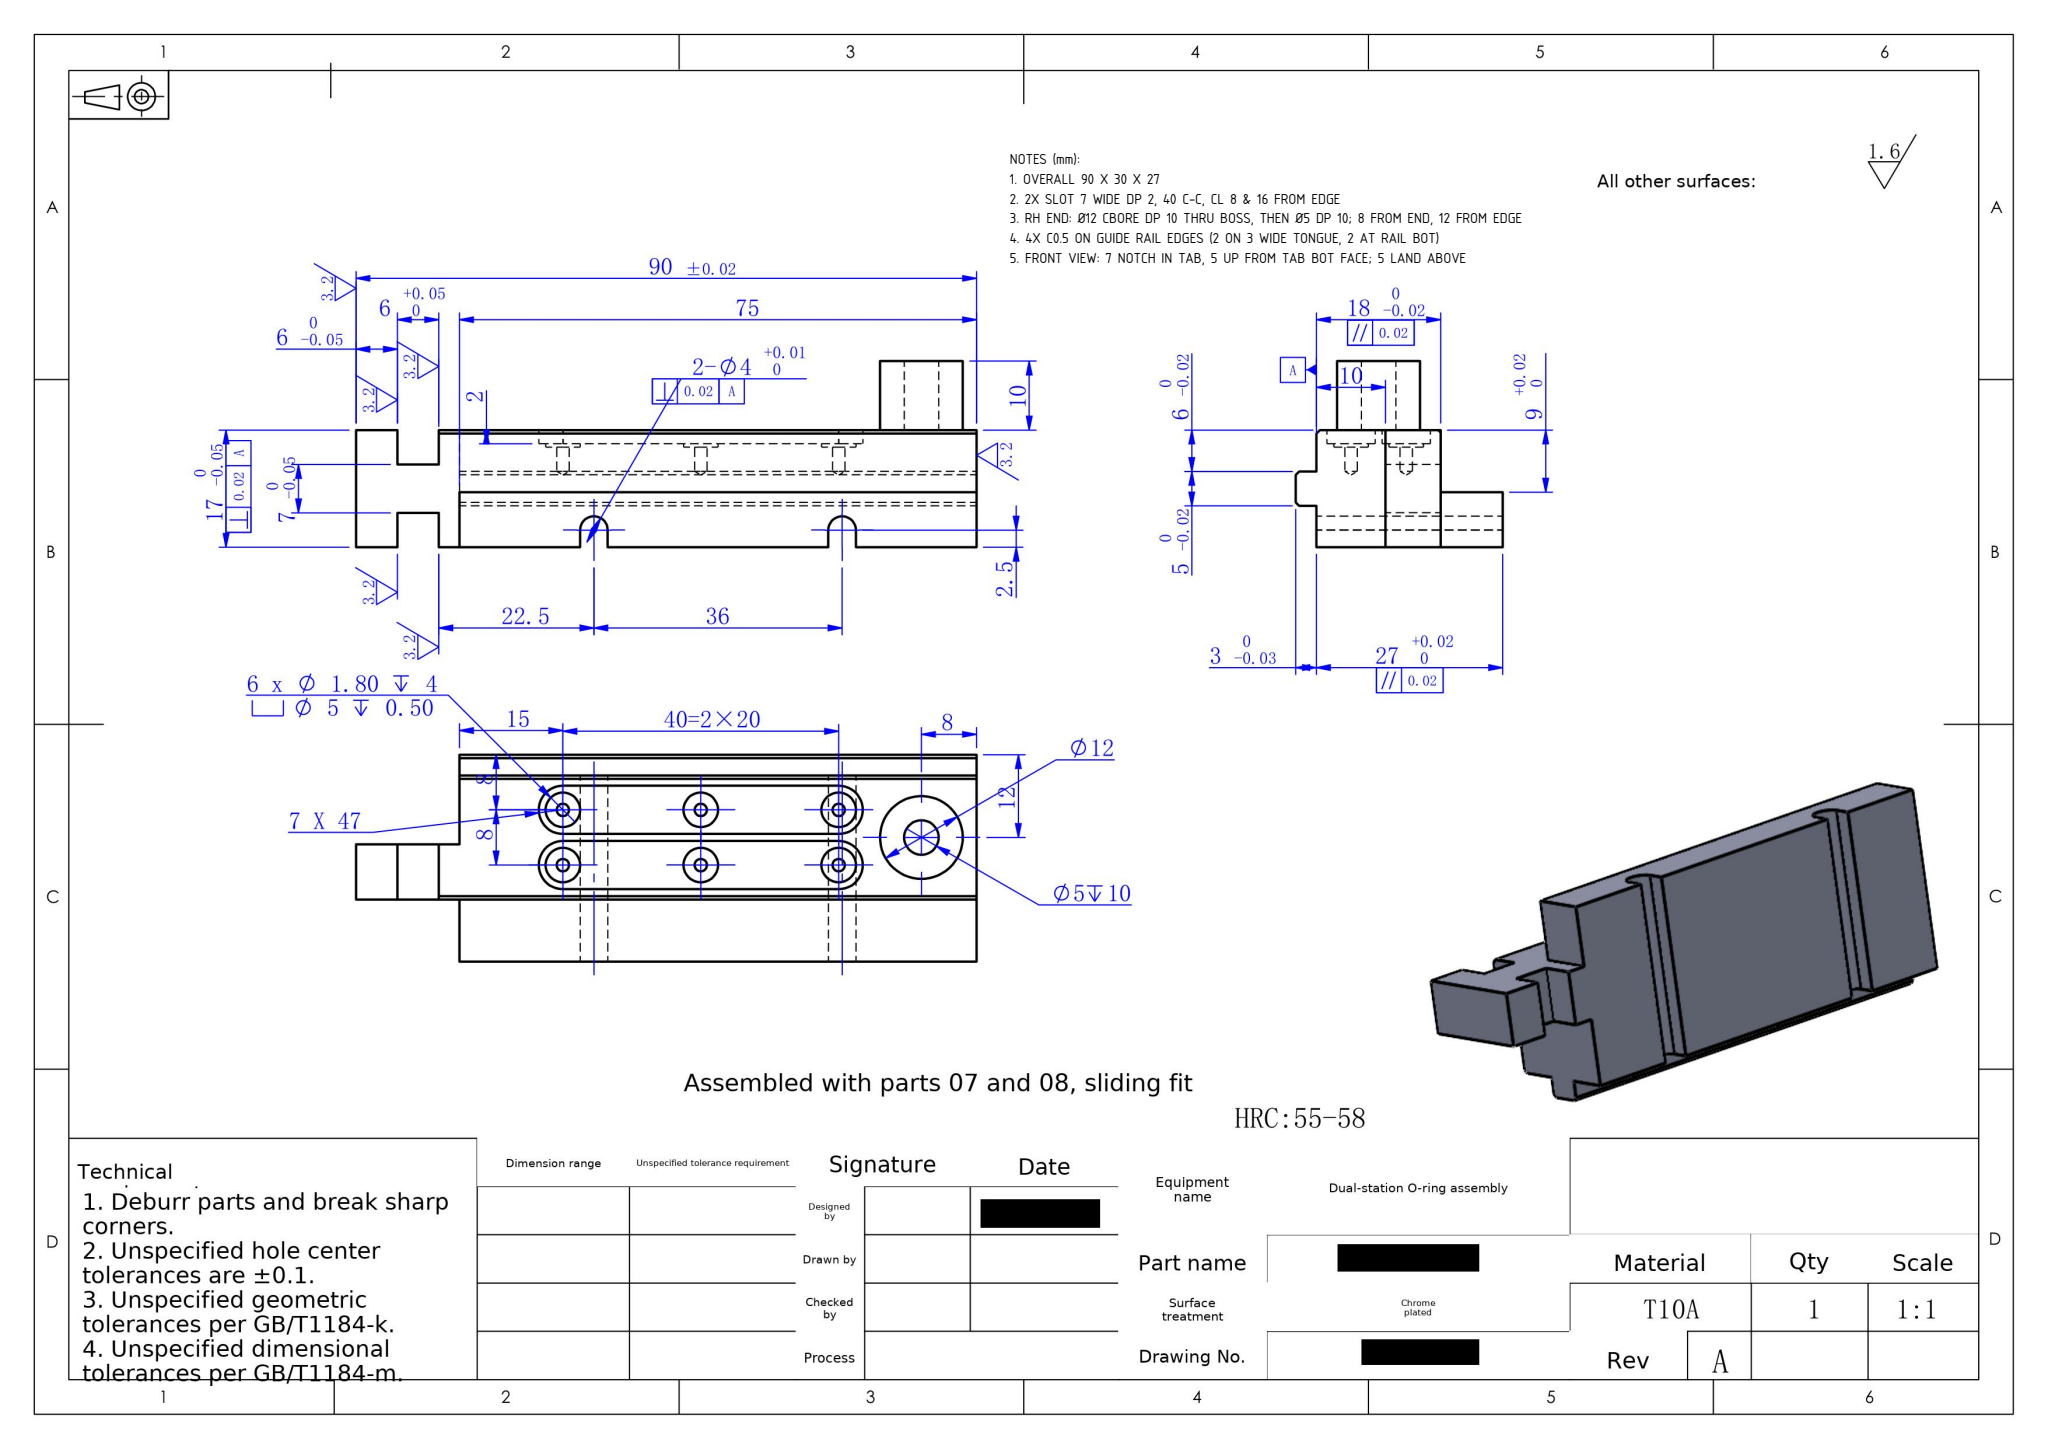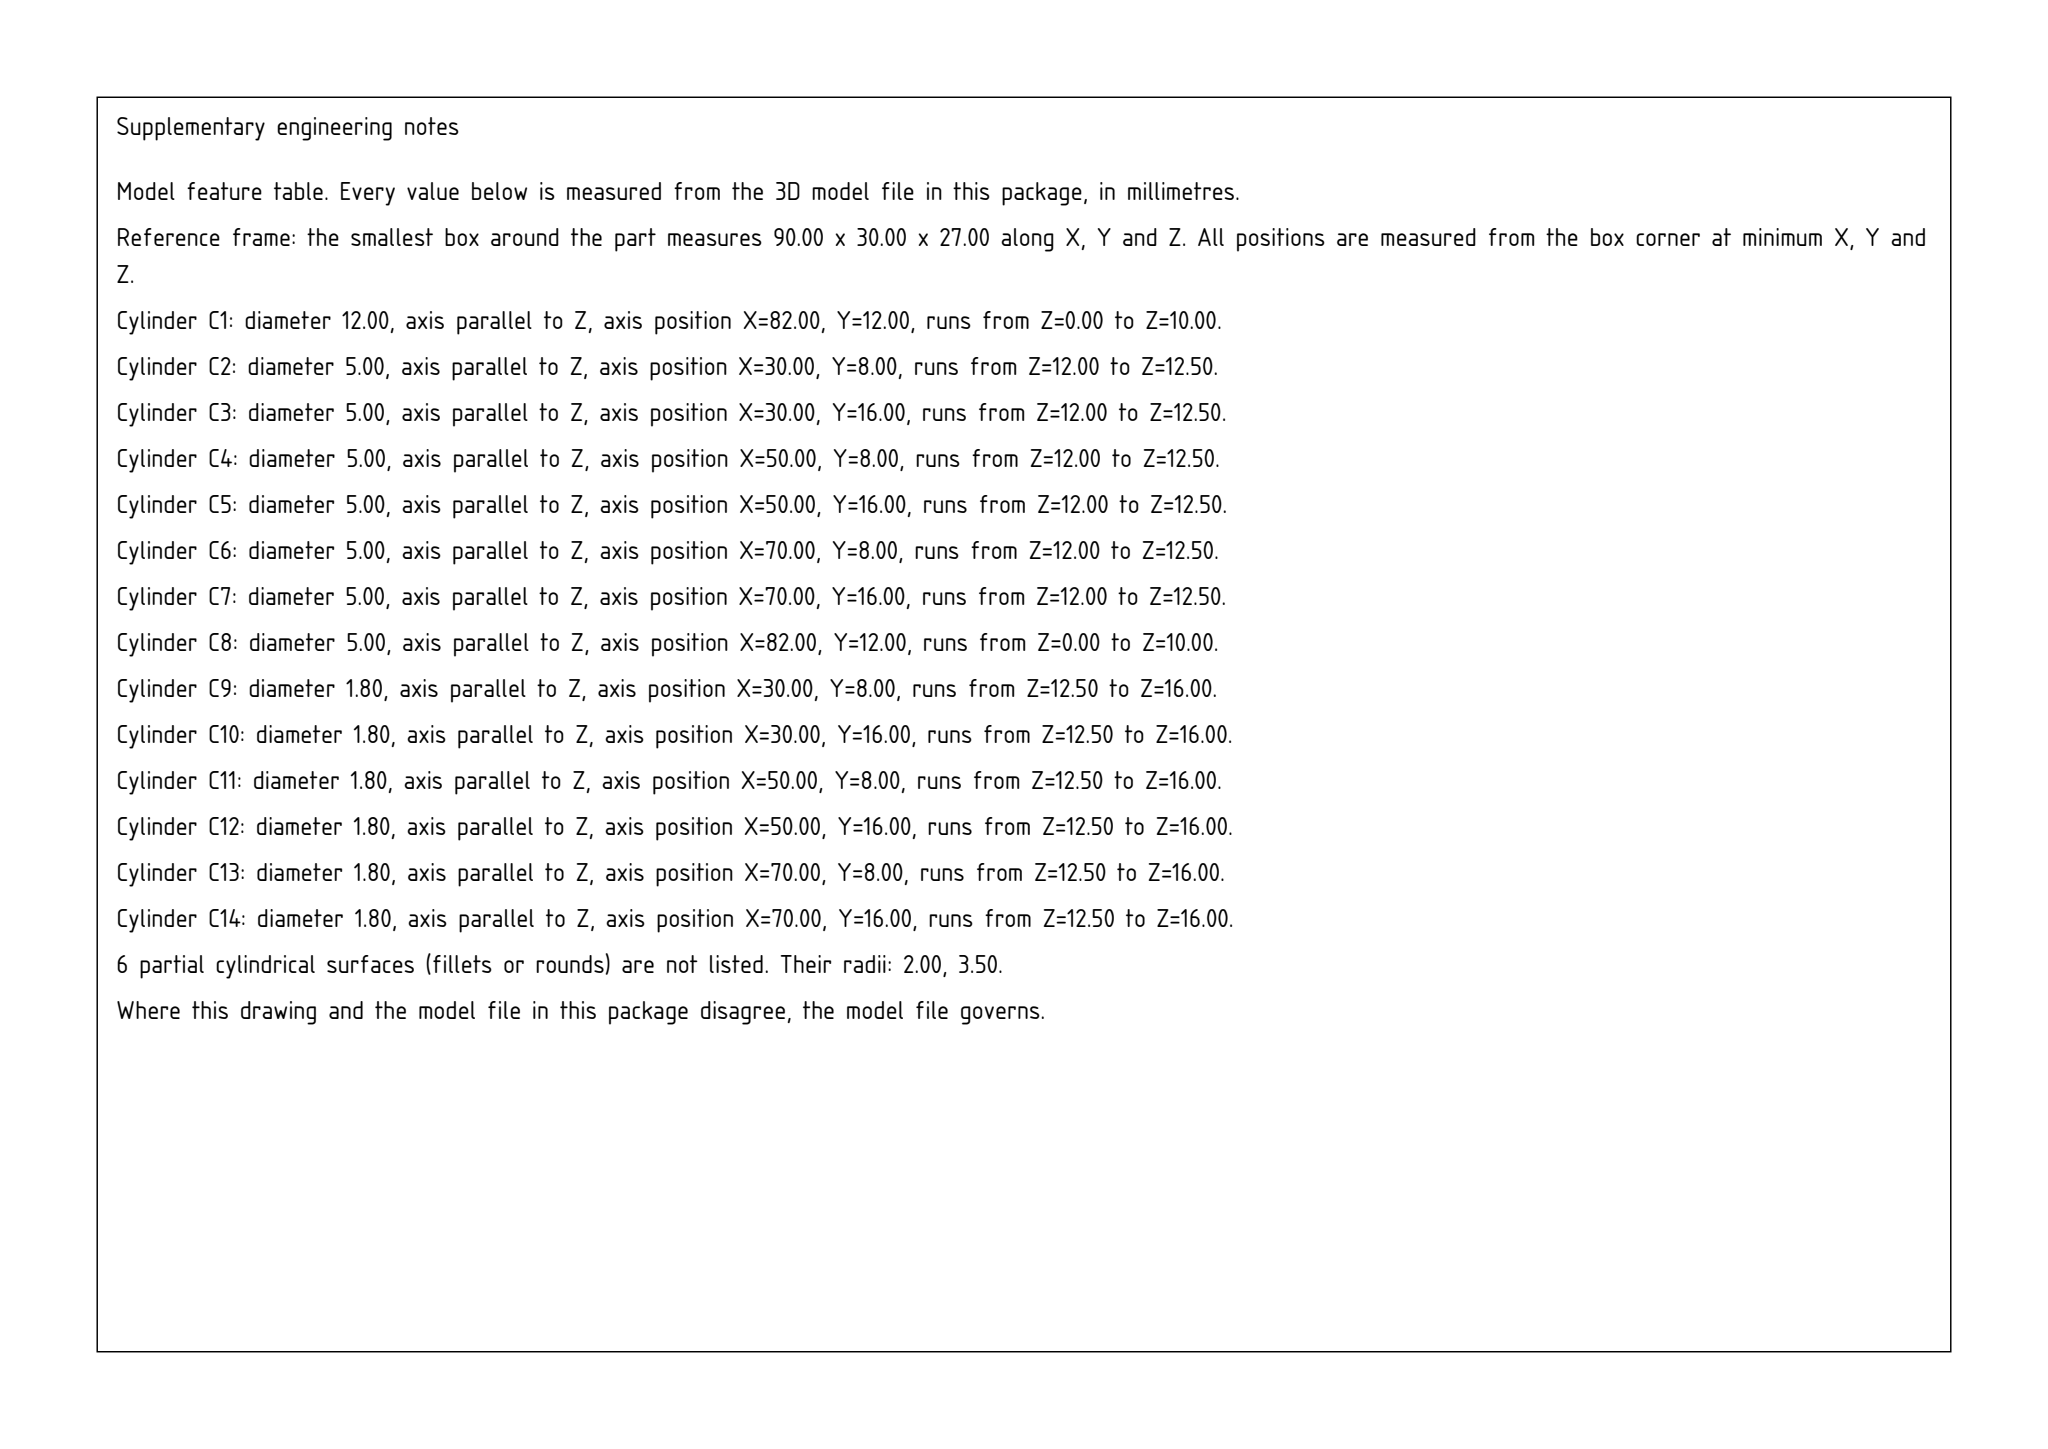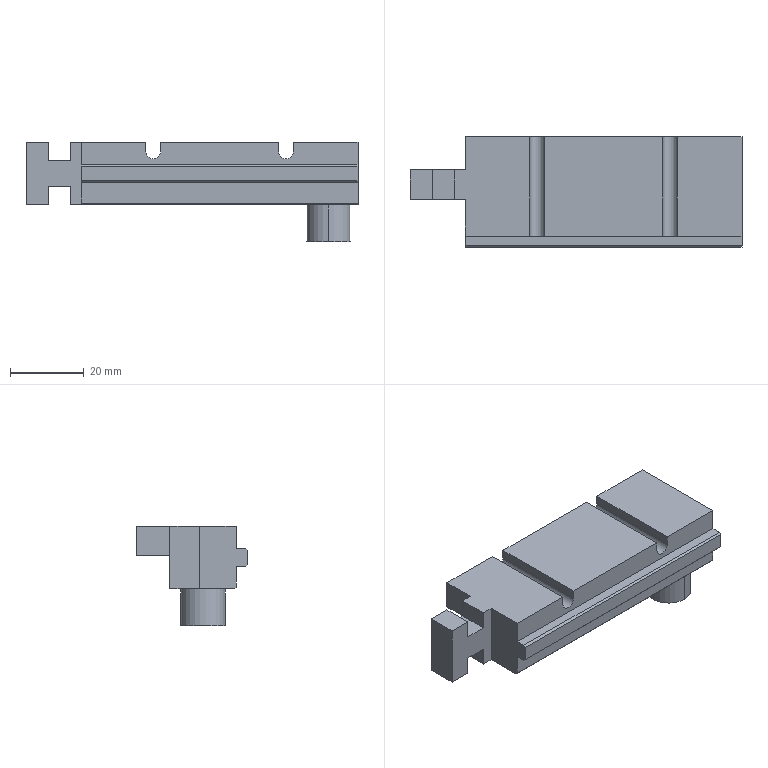Part | SolidWorks | mm | 1 solid | 93 faces | box 90 x 30 x 27 mm | volume 29663 mm3 | plane 47 | cylinder 34 | cone 12 | commonest cylinder face diameters 5 x14 1.8 x12 7 x4 12 x2 4 x2
Drawing notes:
OVERALL 90 X 30 X 27 | from the solid: bbox_xyz [90.0, 30.0, 27.0]
2X SLOT 7 WIDE DP 2, 40 C-C, CL 8 & 16 FROM EDGE | from the solid: 4X Ø7 part-cyl axis z at x=30/70, y=8/16, len 2; slot walls y=4.5/11.5 & 12.5/19.5; bottoms z=12 below top face z=10
RH END: Ø12 CBORE DP 10 THRU BOSS, THEN Ø5 DP 10; 8 FROM END, 12 FROM EDGE | from the solid: cyl [12,z,(82,12),len 10] coaxial with cyl [5,z,(82,12),len 10]; 90-82=8 from RH end, 12 from y=0 edge
4X C0.5 ON GUIDE RAIL EDGES (2 ON 3 WIDE TONGUE, 2 AT RAIL BOT) | from the solid: 4 inclined planes at 45° to y,z, size 0.5x0.5, full length: from [15,0,16], [15,0,20.5] (tongue edges at y=0, z=16 & 20.5), [15,3,10] (lower edge at y=3/z=10) and [12,20.5,10] (lower edge at y=21/z=10)
FRONT VIEW: 7 NOTCH IN TAB, 5 UP FROM TAB BOT FACE; 5 LAND ABOVE | from the solid: X-planes at x=6 & 12, y[13,21], z[10,15] and z[22,27]; tab z 10-27 (17), notch z 15-22 (7), 5 land each side
build123d program:
from build123d import *

# Parameters (mm, degrees)
SKETCH1_W                                            = 75
SKETCH1_H                                            = 27
BOSS_EXTRUDE1_DEPTH                                  = 18
SKETCH4_W                                            = 10
SKETCH4_H                                            = 27
CUT_EXTRUDE2_DEPTH                                   = 94.999
CUT_EXTRUDE3_DEPTH                                   = 90.481
SKETCH7_W                                            = 75
SKETCH7_H                                            = 18
BOSS_EXTRUDE2_DEPTH                                  = 9
SKETCH10_W                                           = 17
SKETCH10_H                                           = 18
BOSS_EXTRUDE4_DEPTH                                  = 15
SKETCH11_W                                           = 6
SKETCH11_H                                           = 5
CUT_EXTRUDE4_DEPTH                                   = 102.63
CHAMFER2_SIZE                                        = 0.5
SKETCH12_W                                           = 5
SKETCH12_H                                           = 3
BOSS_EXTRUDE5_DEPTH                                  = 75
SKETCH13_W                                           = 12
SKETCH13_H                                           = 10
CUT_EXTRUDE5_DEPTH                                   = 114.386
CHAMFER3_SIZE                                        = 0.5
SKETCH14_W                                           = 3
SKETCH14_H                                           = 17
CUT_EXTRUDE6_DEPTH                                   = 10
SKETCH15_R                                           = 6
SKETCH15_R_2                                         = 2.5
BOSS_EXTRUDE6_DEPTH                                  = 10
CUT_EXTRUDE7_DEPTH                                   = 2
CYLINDRICAL_COUNTERSUNK_HOLE_FOR_M1_6_HE_D           = 1.8
CYLINDRICAL_COUNTERSUNK_HOLE_FOR_M1_6_HE_DEPTH       = 4
CYLINDRICAL_COUNTERSUNK_HOLE_FOR_M1_6_HE_CBORE_D     = 5
CYLINDRICAL_COUNTERSUNK_HOLE_FOR_M1_6_HE_CBORE_DEPTH = 0.5
CYLINDRICAL_COUNTERSUNK_HOLE_FOR_M1_6_HE_TIP         = 0.5408


with BuildPart() as part:
    # Sketch1 → Boss-Extrude1 (new body)
    with BuildSketch(Plane.XY):
        with Locations((-45.89, 40.229)):
            Rectangle(SKETCH1_W, SKETCH1_H)
    extrude(amount=BOSS_EXTRUDE1_DEPTH)

    # Sketch4 → Cut-Extrude2 (cut, through all)
    with BuildSketch(Plane.ZY.offset(83.39)):
        with Locations((5, 40.229)):
            Rectangle(SKETCH4_W, SKETCH4_H)
    extrude(amount=-CUT_EXTRUDE2_DEPTH, mode=Mode.SUBTRACT)

    # Sketch5 → Cut-Extrude3 (cut, through all)
    with BuildSketch(Plane(origin=(0, 53.729, 0), x_dir=(1, 0, 0), z_dir=(0, 1, 0))):
        with BuildLine():
            Line((-65.89, -15.5), (-65.89, -18))
            Line((-65.89, -18), (-61.89, -18))
            Line((-61.89, -18), (-61.89, -15.5))
            ThreePointArc((-61.89, -15.5), (-63.89, -13.5), (-65.89, -15.5))
        make_face()
        with BuildLine():
            Line((-25.89, -18), (-29.89, -18))
            Line((-29.89, -18), (-29.89, -15.5))
            ThreePointArc((-29.89, -15.5), (-27.89, -13.5), (-25.89, -15.5))
            Line((-25.89, -15.5), (-25.89, -18))
        make_face()
    extrude(amount=-CUT_EXTRUDE3_DEPTH, mode=Mode.SUBTRACT)

    # Sketch7 → Boss-Extrude2 (add)
    with BuildSketch(Plane(origin=(0, 0, 10), x_dir=(-1, 0, 0), z_dir=(0, 0, -1))):
        with Locations((45.89, 35.729)):
            Rectangle(SKETCH7_W, SKETCH7_H)
    extrude(amount=BOSS_EXTRUDE2_DEPTH)

    # Sketch10 → Boss-Extrude4 (add)
    with BuildSketch(Plane.ZY.offset(83.39)):
        with Locations((9.5, 35.729)):
            Rectangle(SKETCH10_W, SKETCH10_H)
    extrude(amount=BOSS_EXTRUDE4_DEPTH)

    # Sketch11 → Cut-Extrude4 (cut, through all)
    with BuildSketch(Plane(origin=(0, 44.729, 0), x_dir=(1, 0, 0), z_dir=(0, 1, 0))):
        with Locations((-89.39, -3.5)):
            Rectangle(SKETCH11_W, SKETCH11_H)
        with Locations((-89.39, -15.5)):
            Rectangle(SKETCH11_W, SKETCH11_H)
    extrude(amount=-CUT_EXTRUDE4_DEPTH, mode=Mode.SUBTRACT)

    # Chamfer2
    chamfer2_edges = [part.edges().sort_by_distance(p)[0] for p in [
        (-47.39, 26.729, 1),
    ]]
    chamfer(chamfer2_edges, length=CHAMFER2_SIZE)

    # Sketch12 → Boss-Extrude5 (add)
    with BuildSketch(Plane(origin=(-8.39, 0, 0), x_dir=(0, 0, -1), z_dir=(1, 0, 0))):
        with Locations((-9.5, 25.229)):
            Rectangle(SKETCH12_W, SKETCH12_H)
    extrude(amount=-BOSS_EXTRUDE5_DEPTH)

    # Sketch13 → Cut-Extrude5 (cut, through all)
    with BuildSketch(Plane(origin=(0, 0, 1), x_dir=(-1, 0, 0), z_dir=(0, 0, -1))):
        with Locations((92.39, 31.729)):
            Rectangle(SKETCH13_W, SKETCH13_H)
    extrude(amount=-CUT_EXTRUDE5_DEPTH, mode=Mode.SUBTRACT)

    # Chamfer3
    chamfer3_edges = [part.edges().sort_by_distance(p)[0] for p in [
        (-45.89, 23.729, 12),
        (-45.89, 23.729, 7),
        (-47.39, 44.729, 1),
    ]]
    chamfer(chamfer3_edges, length=CHAMFER3_SIZE)

    # Sketch14 → Cut-Extrude6 (cut)
    with BuildSketch(Plane.XZ.offset(-26.729)):
        with Locations((-84.89, 9.5)):
            Rectangle(SKETCH14_W, SKETCH14_H)
    extrude(amount=-CUT_EXTRUDE6_DEPTH, mode=Mode.SUBTRACT)

    # Sketch15 → Boss-Extrude6 (add)
    with BuildSketch(Plane(origin=(0, 0, 1), x_dir=(-1, 0, 0), z_dir=(0, 0, -1))):
        with Locations(Location((16.39, 35.729, 0), (0, 0, 270))):
            Circle(SKETCH15_R)
        with Locations(Location((16.39, 35.729, 0), (0, 0, 90))):
            Circle(SKETCH15_R_2, mode=Mode.SUBTRACT)
    extrude(amount=BOSS_EXTRUDE6_DEPTH)

    # Sketch16 → Cut-Extrude7 (cut)
    with BuildSketch(Plane(origin=(0, 0, 1), x_dir=(-1, 0, 0), z_dir=(0, 0, -1))):
        with BuildLine():
            Line((28.39, 43.229), (68.39, 43.229))
            ThreePointArc((68.39, 43.229), (71.89, 39.729), (68.39, 36.229))
            Line((68.39, 36.229), (28.39, 36.229))
            ThreePointArc((28.39, 36.229), (24.89, 39.729), (28.39, 43.229))
        make_face()
        with BuildLine():
            Line((28.39, 35.229), (68.39, 35.229))
            ThreePointArc((68.39, 35.229), (71.89, 31.729), (68.39, 28.229))
            Line((68.39, 28.229), (28.39, 28.229))
            ThreePointArc((28.39, 28.229), (24.89, 31.729), (28.39, 35.229))
        make_face()
    extrude(amount=-CUT_EXTRUDE7_DEPTH, mode=Mode.SUBTRACT)

    # Cylindrical Countersunk Hole for M1.6 He
    with Locations(Plane(origin=(0, 0, 3), x_dir=(-1, 0, 0), z_dir=(0, 0, -1))):
        with Locations((28.39, 39.729), (68.39, 39.729), (28.39, 31.729), (68.39, 31.729), (48.39, 39.729), (48.39, 31.729)):
            CounterBoreHole(CYLINDRICAL_COUNTERSUNK_HOLE_FOR_M1_6_HE_D / 2, CYLINDRICAL_COUNTERSUNK_HOLE_FOR_M1_6_HE_CBORE_D / 2, CYLINDRICAL_COUNTERSUNK_HOLE_FOR_M1_6_HE_CBORE_DEPTH, depth=CYLINDRICAL_COUNTERSUNK_HOLE_FOR_M1_6_HE_DEPTH)
            with Locations((0, 0, -(CYLINDRICAL_COUNTERSUNK_HOLE_FOR_M1_6_HE_DEPTH + CYLINDRICAL_COUNTERSUNK_HOLE_FOR_M1_6_HE_TIP / 2))):  # 118° drill point
                Cone(0, CYLINDRICAL_COUNTERSUNK_HOLE_FOR_M1_6_HE_D / 2, CYLINDRICAL_COUNTERSUNK_HOLE_FOR_M1_6_HE_TIP, mode=Mode.SUBTRACT)


solid = part.part